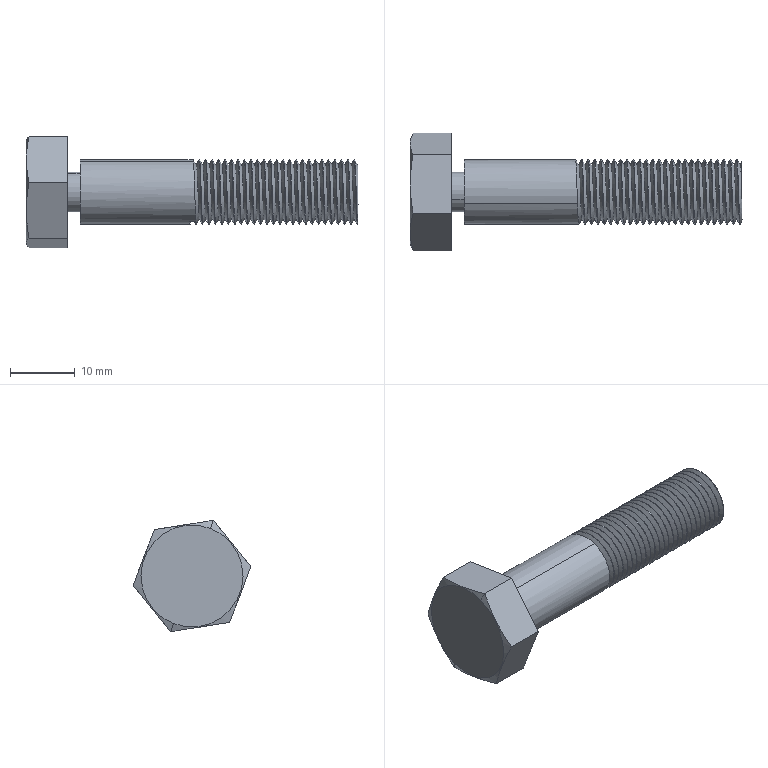Component | SolidWorks | UpperHousingAssembly-1_M10-45-1 | 1 solid | 71 faces | volume 4563 mm3 | cylinder 55 | plane 12 | cone 2 | spline 2 | commonest cylinder face diameters 10 x53 6.183 x2